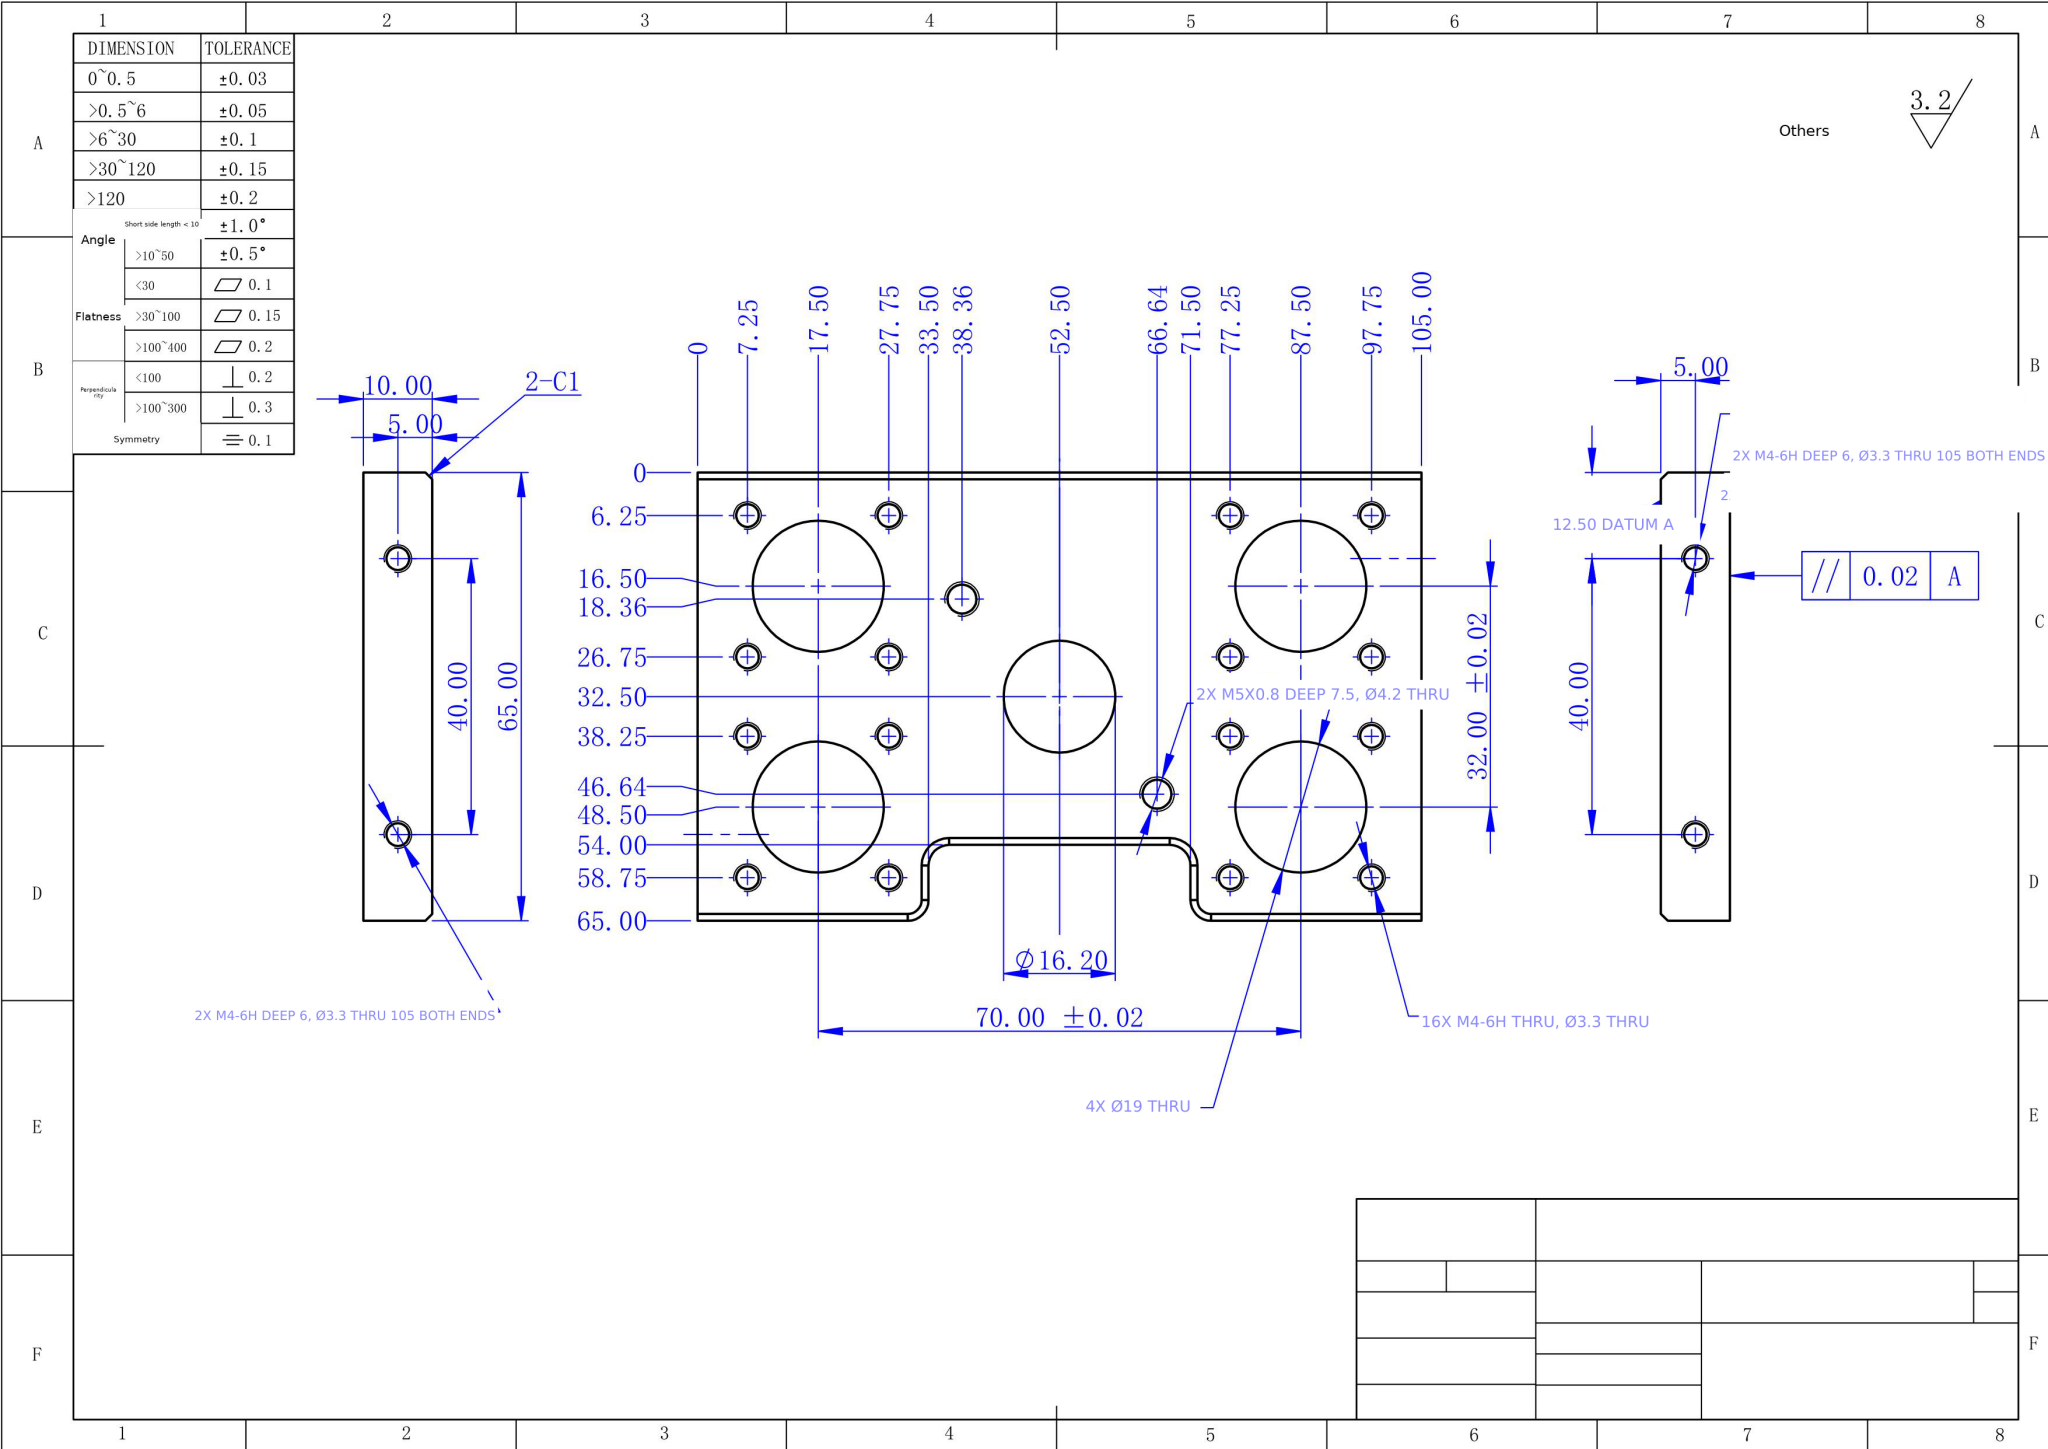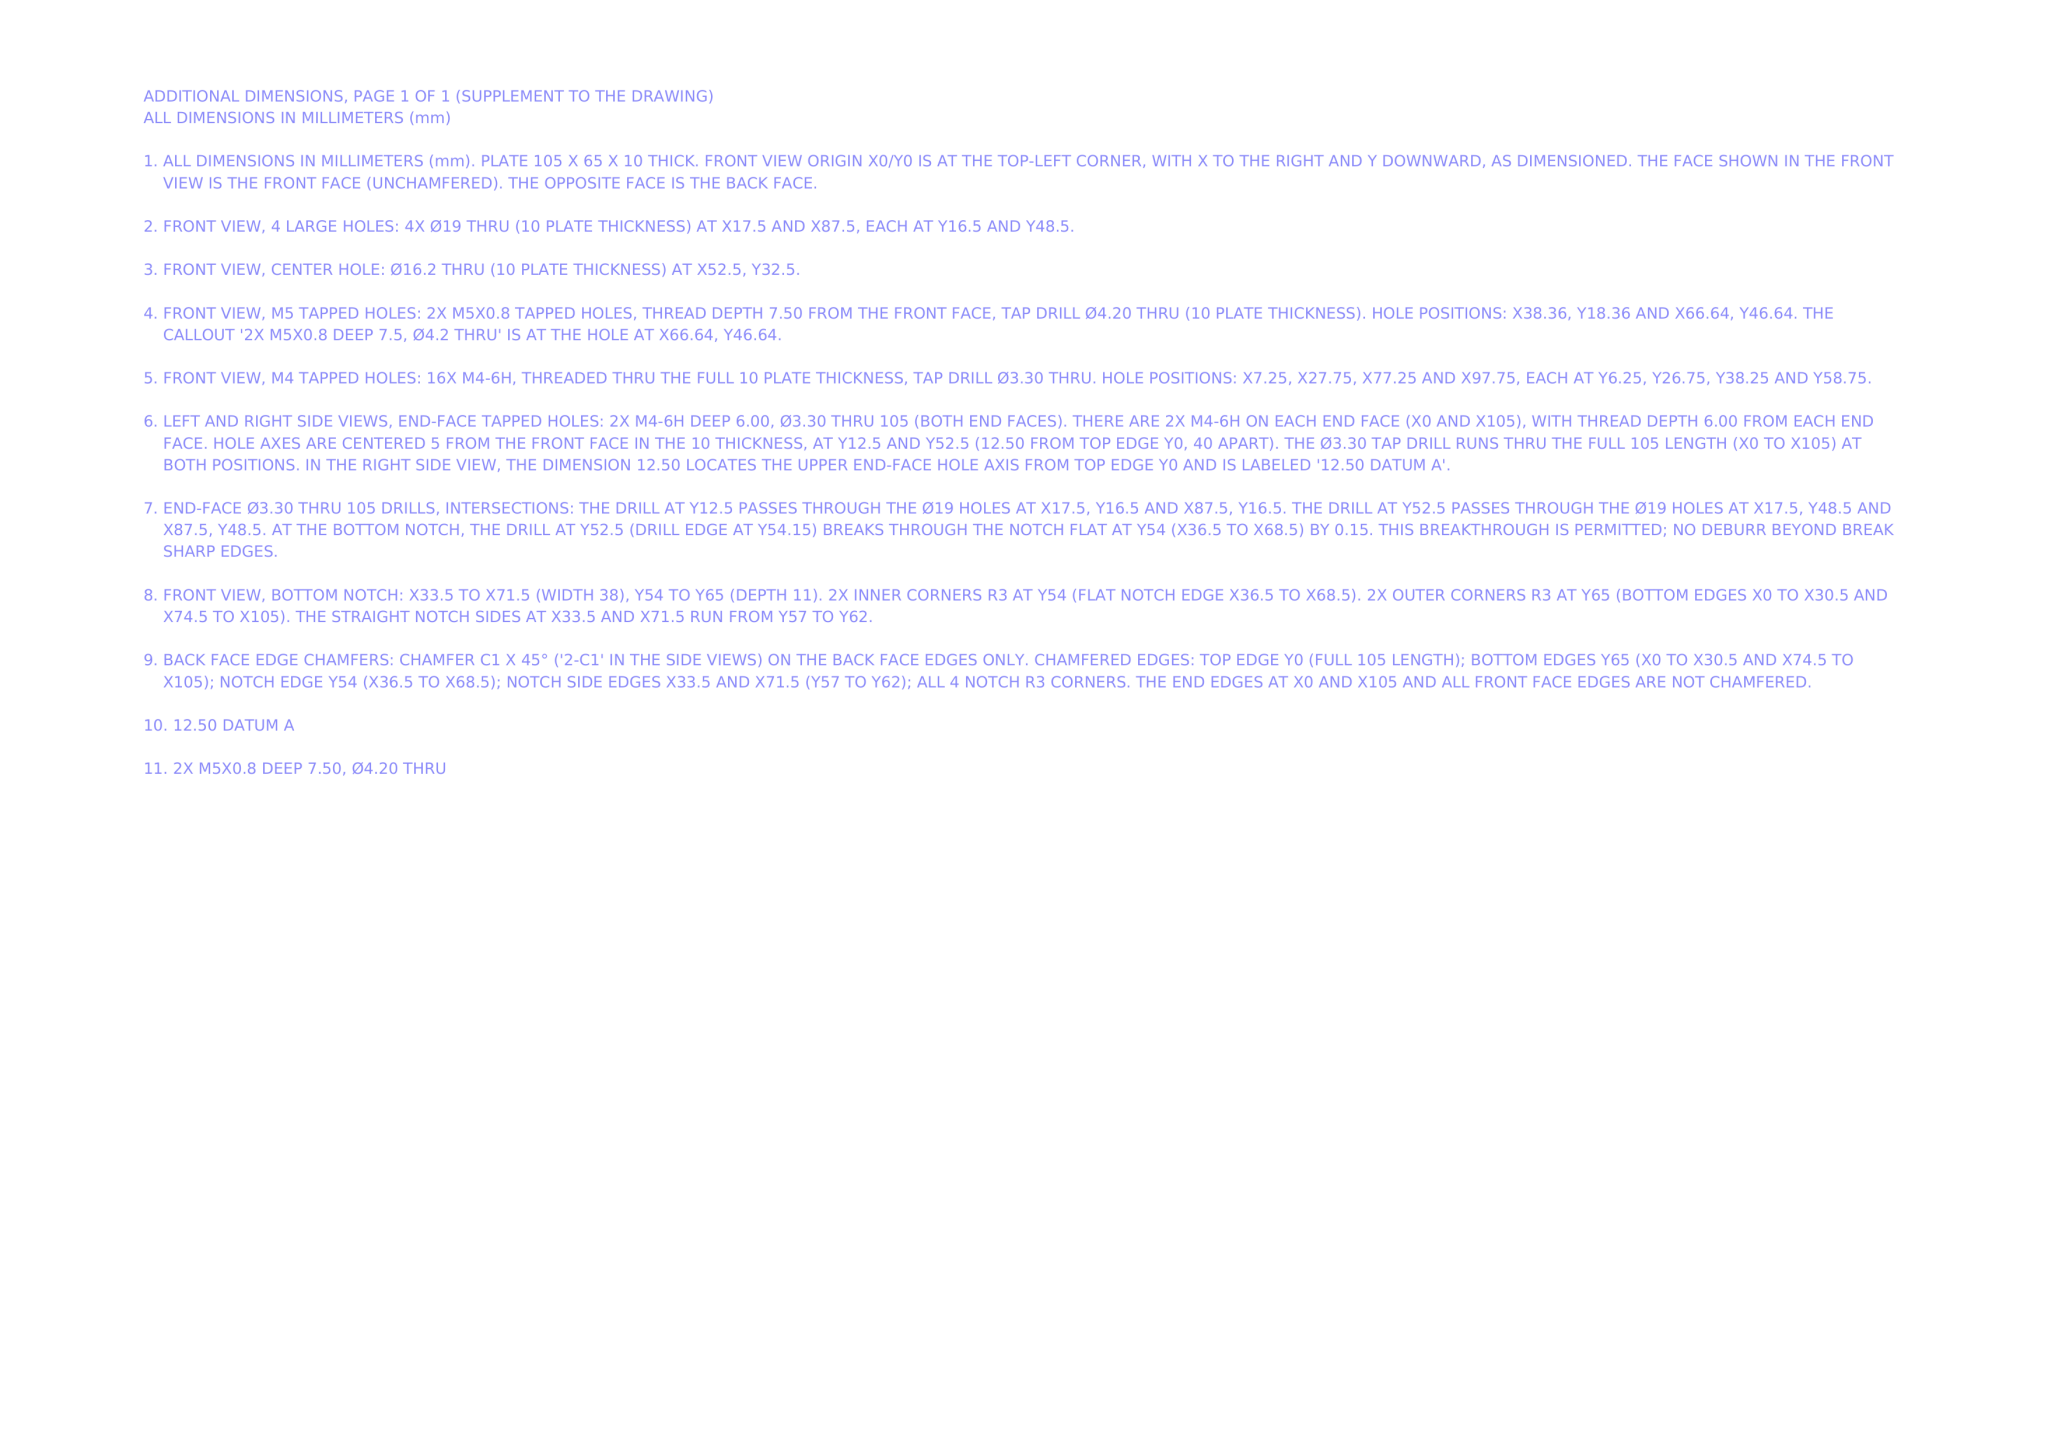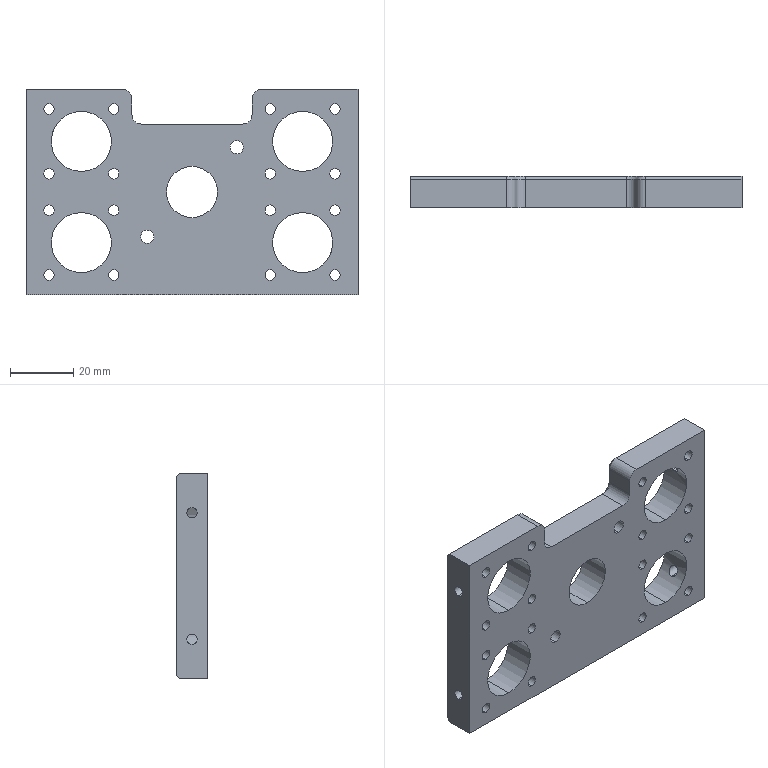Part | NX | mm | 1 solid | 78 faces | box 105 x 10 x 65 mm | volume 48603 mm3 | cylinder 58 | plane 16 | cone 4 | commonest cylinder face diameters 3.3 x40 19 x8 4.2 x4 6 x4 16.2 x2